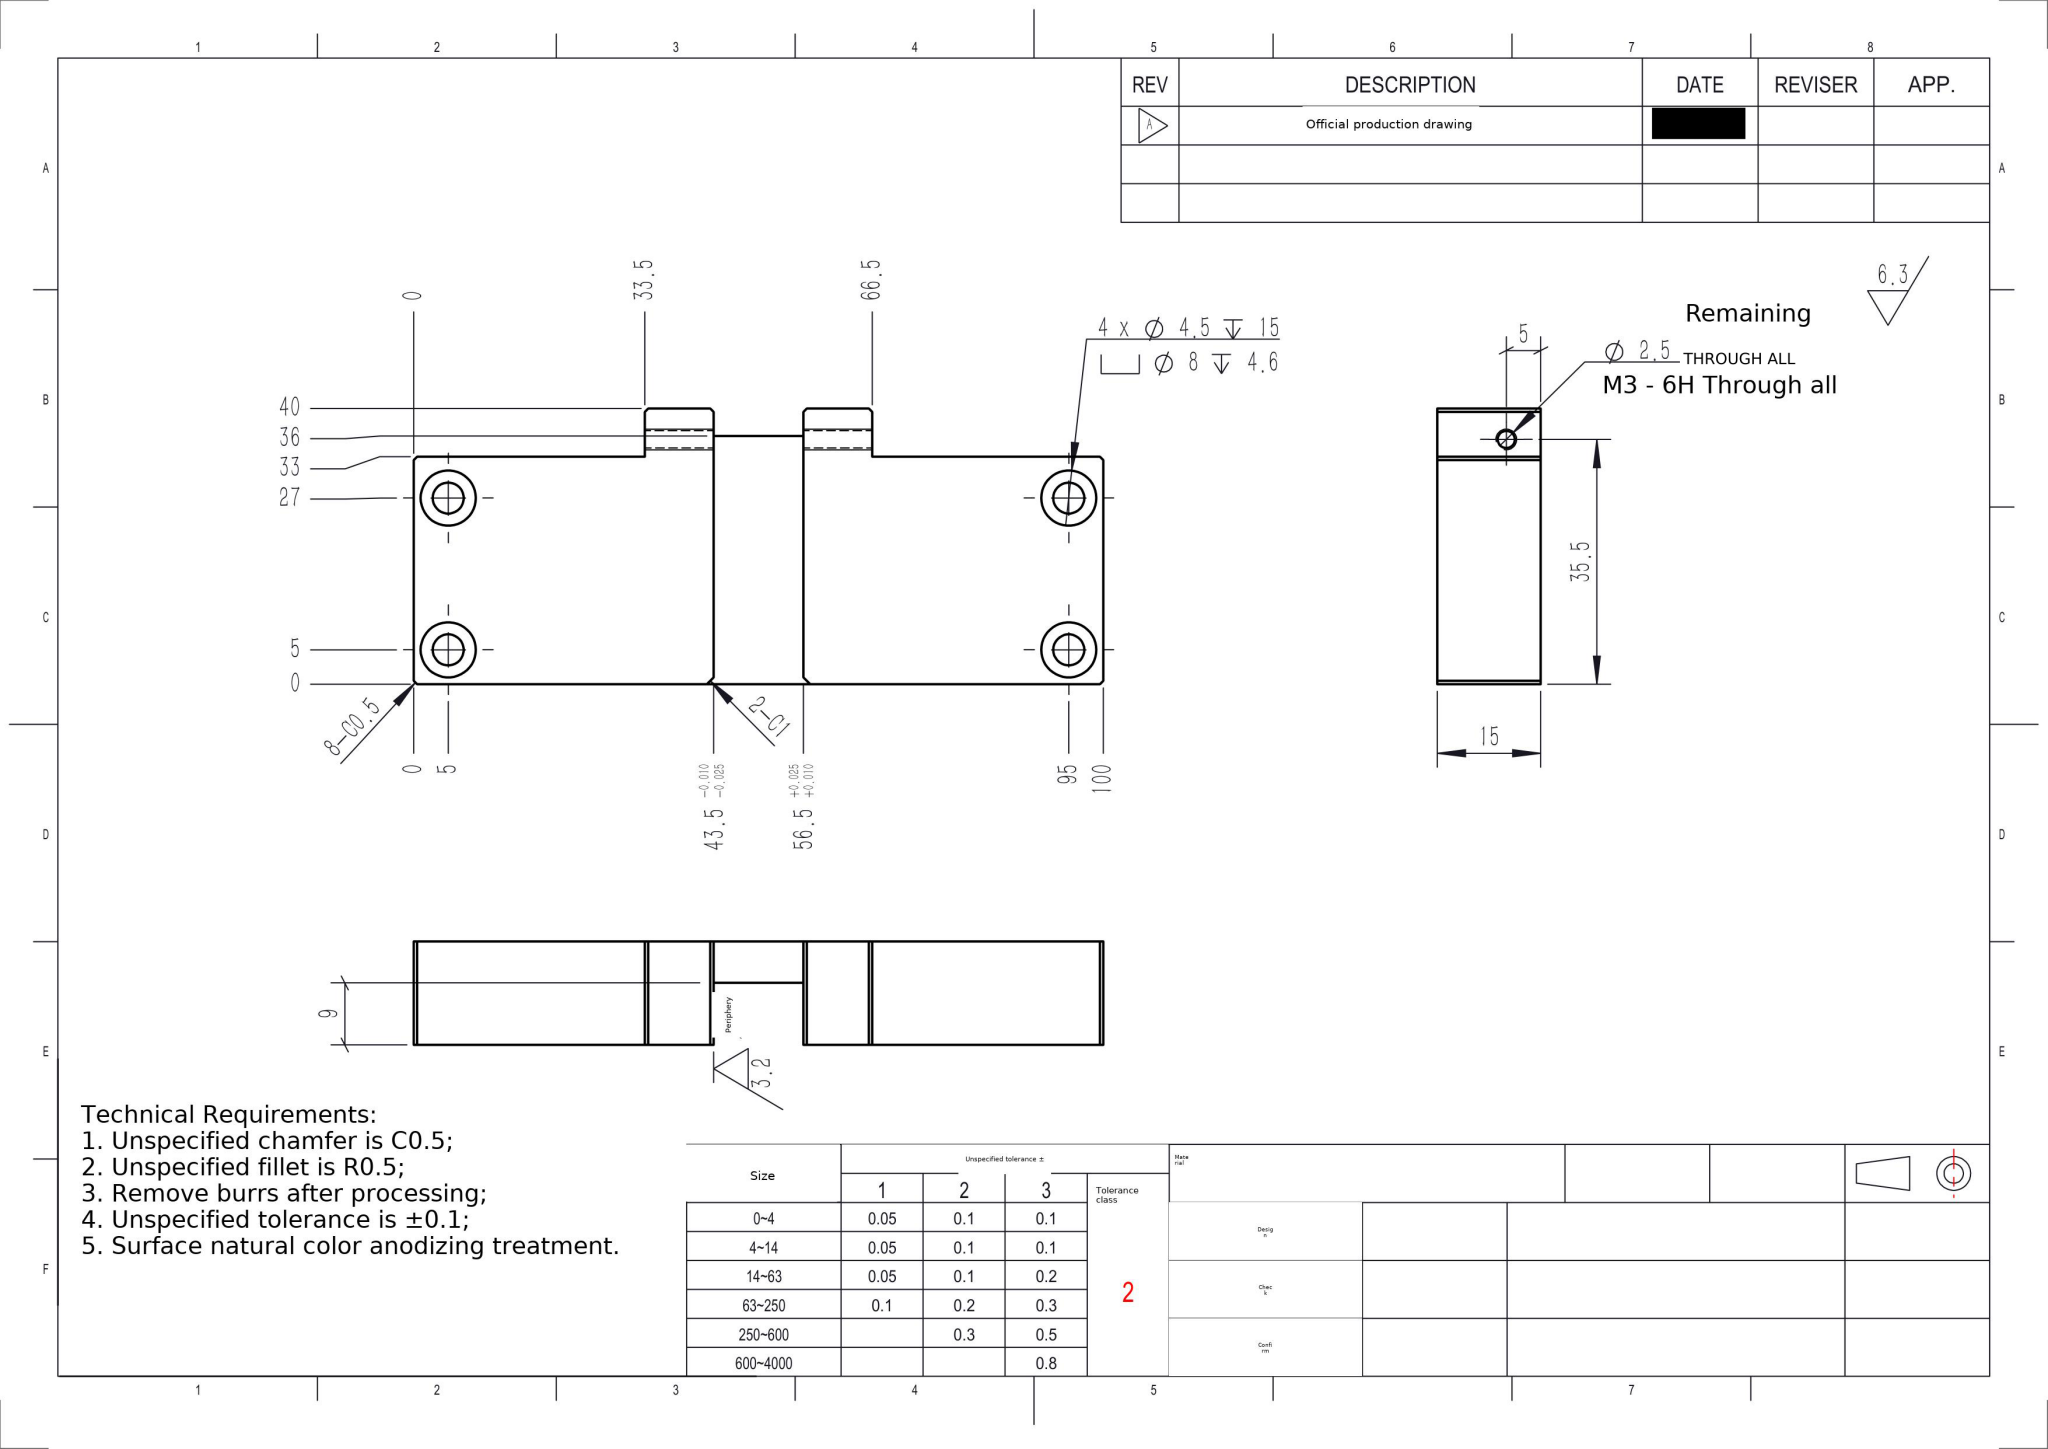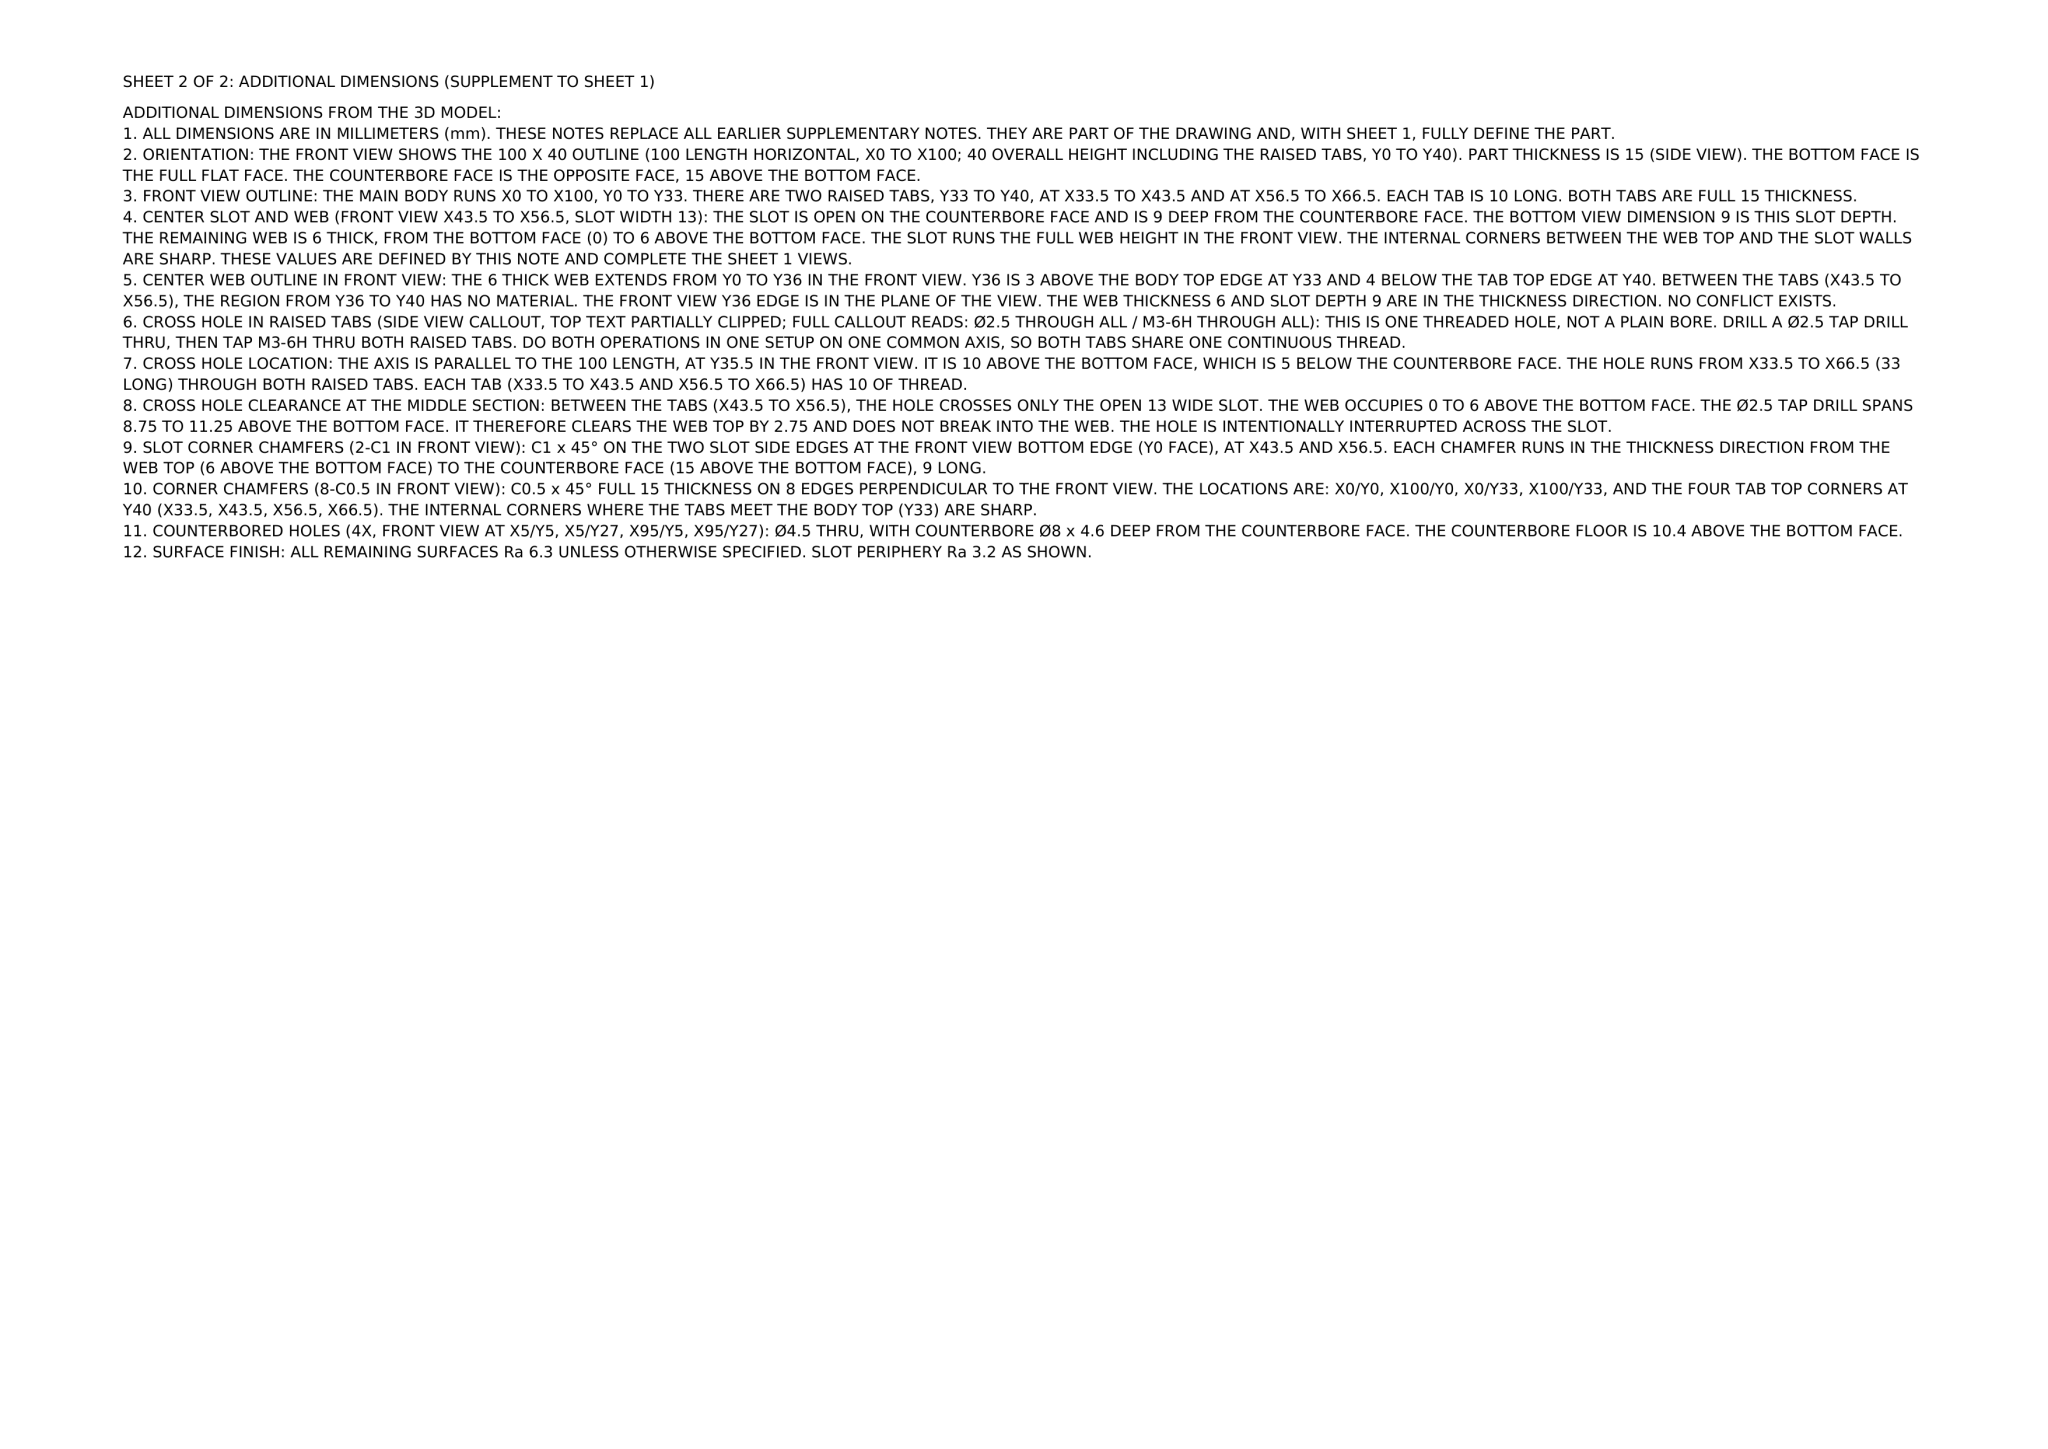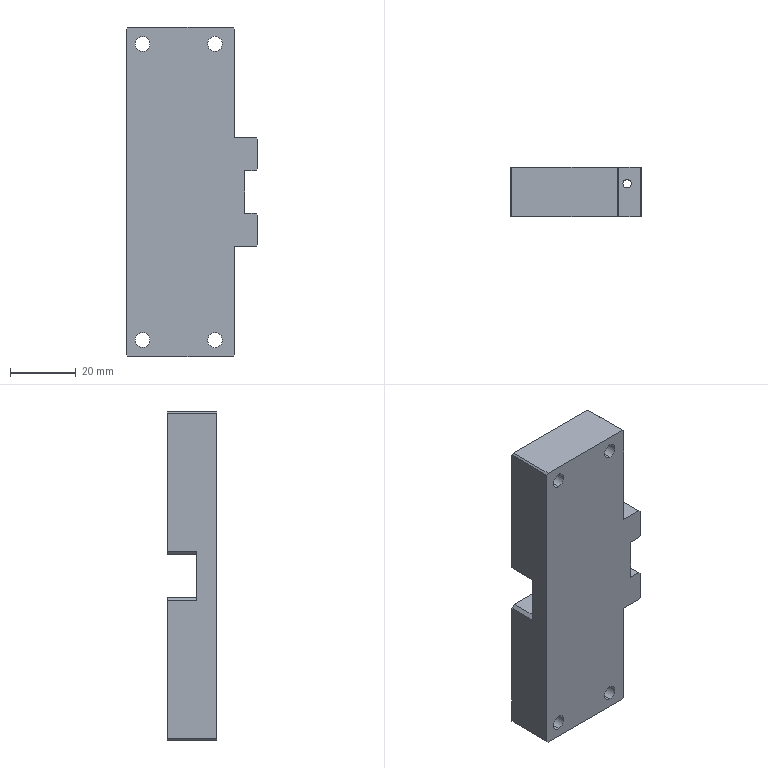Part | NX | mm | 1 solid | 50 faces | box 40 x 15 x 100 mm | volume 46264 mm3 | plane 30 | cylinder 20 | commonest cylinder face diameters 8 x8 4.5 x8 2.5 x4